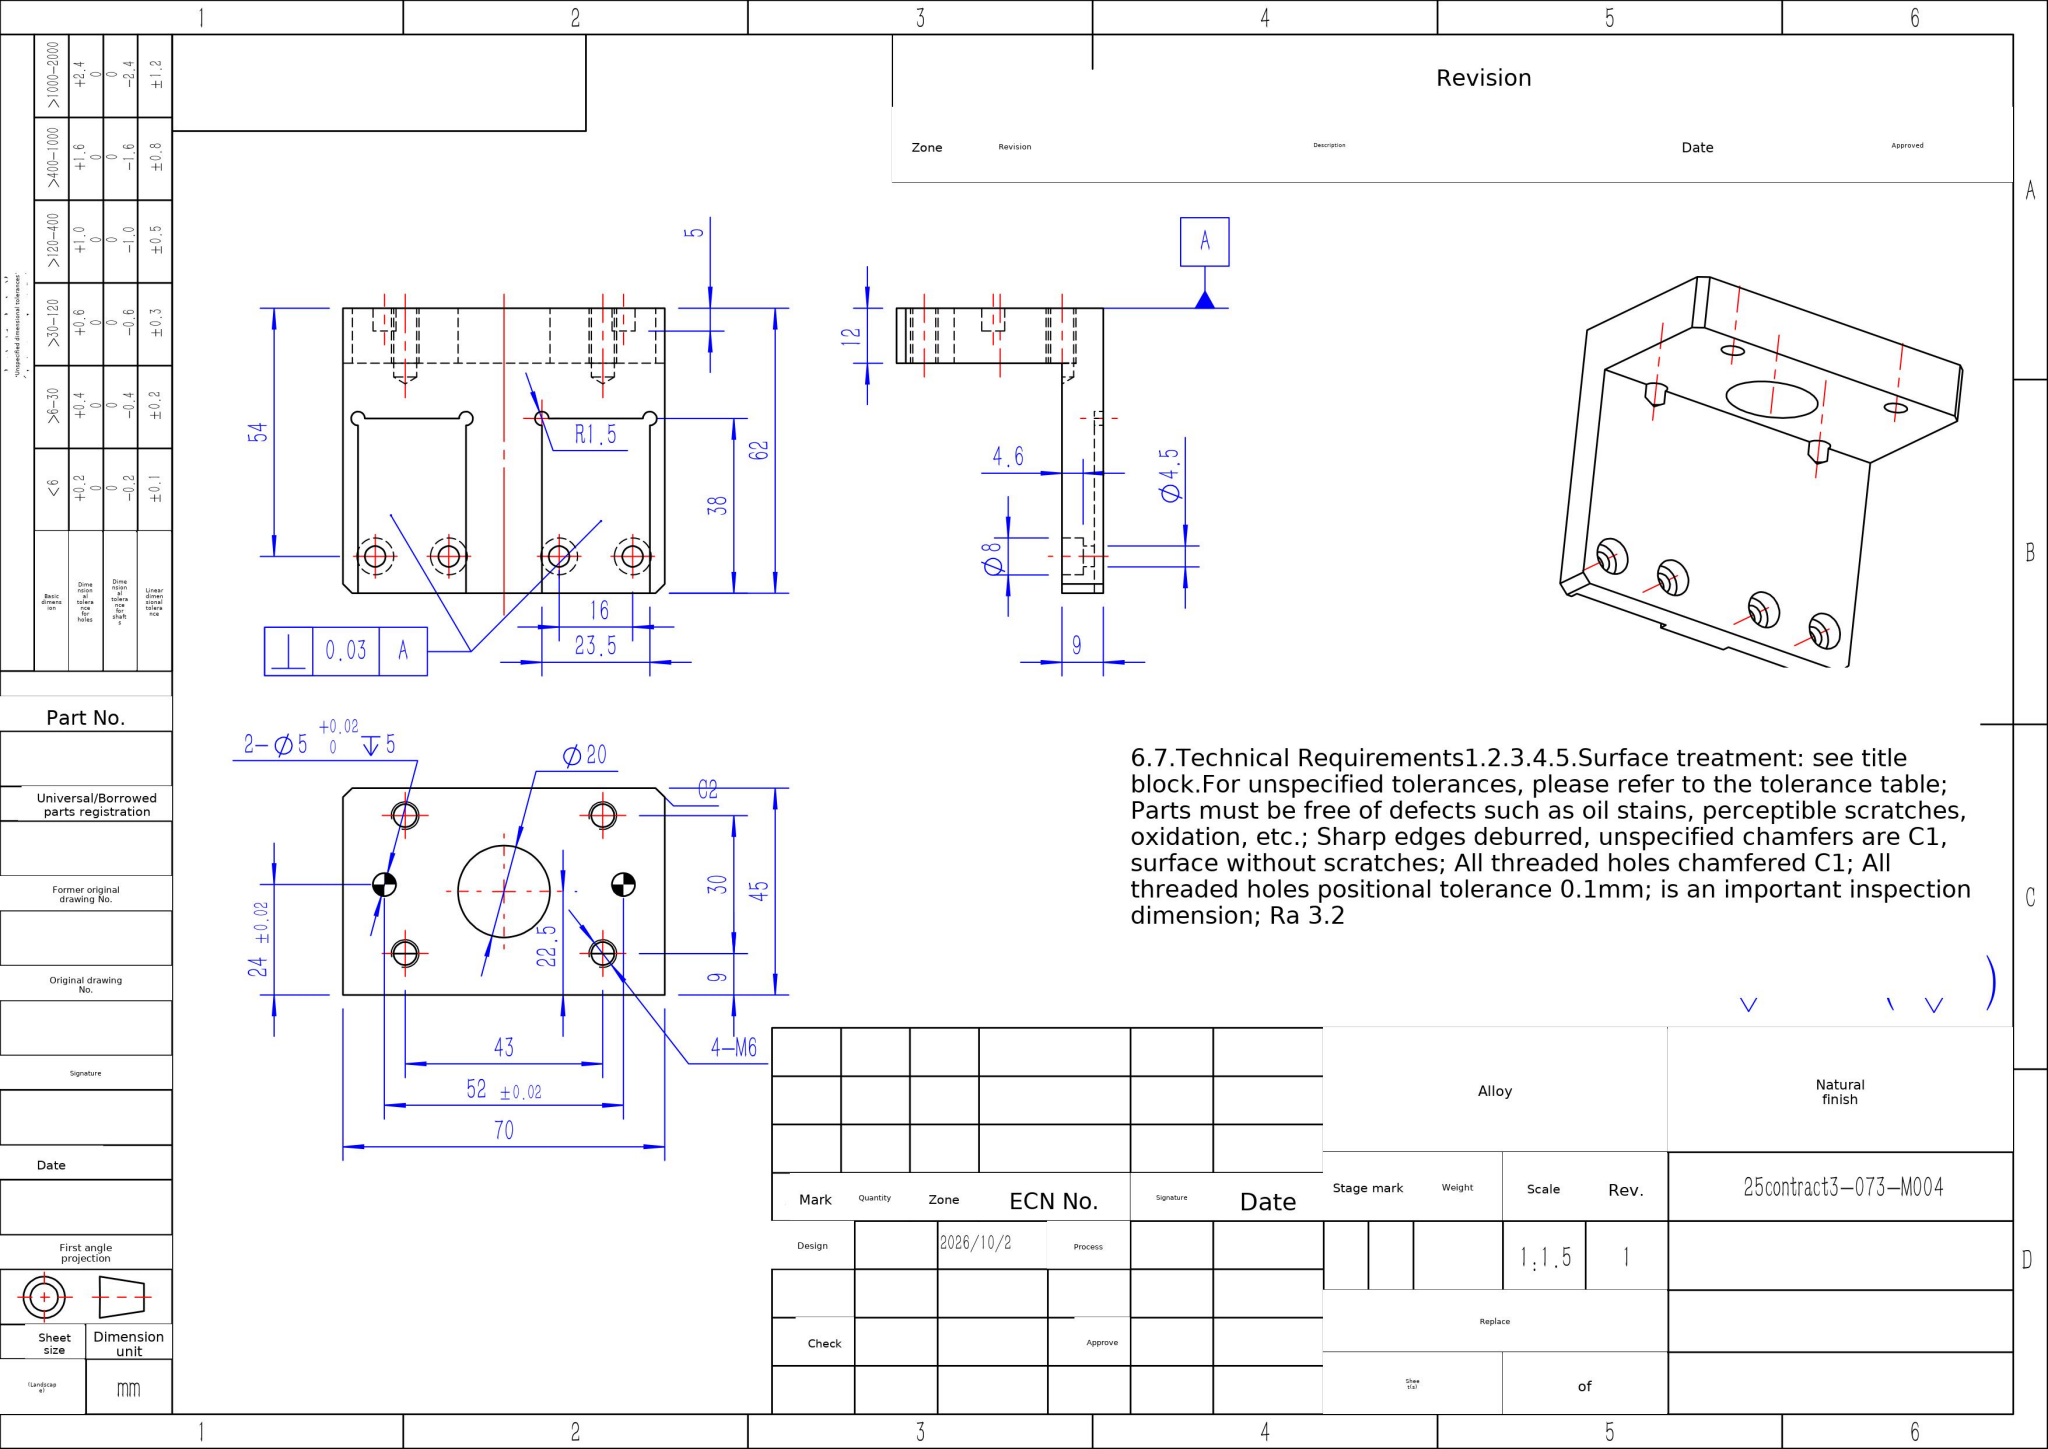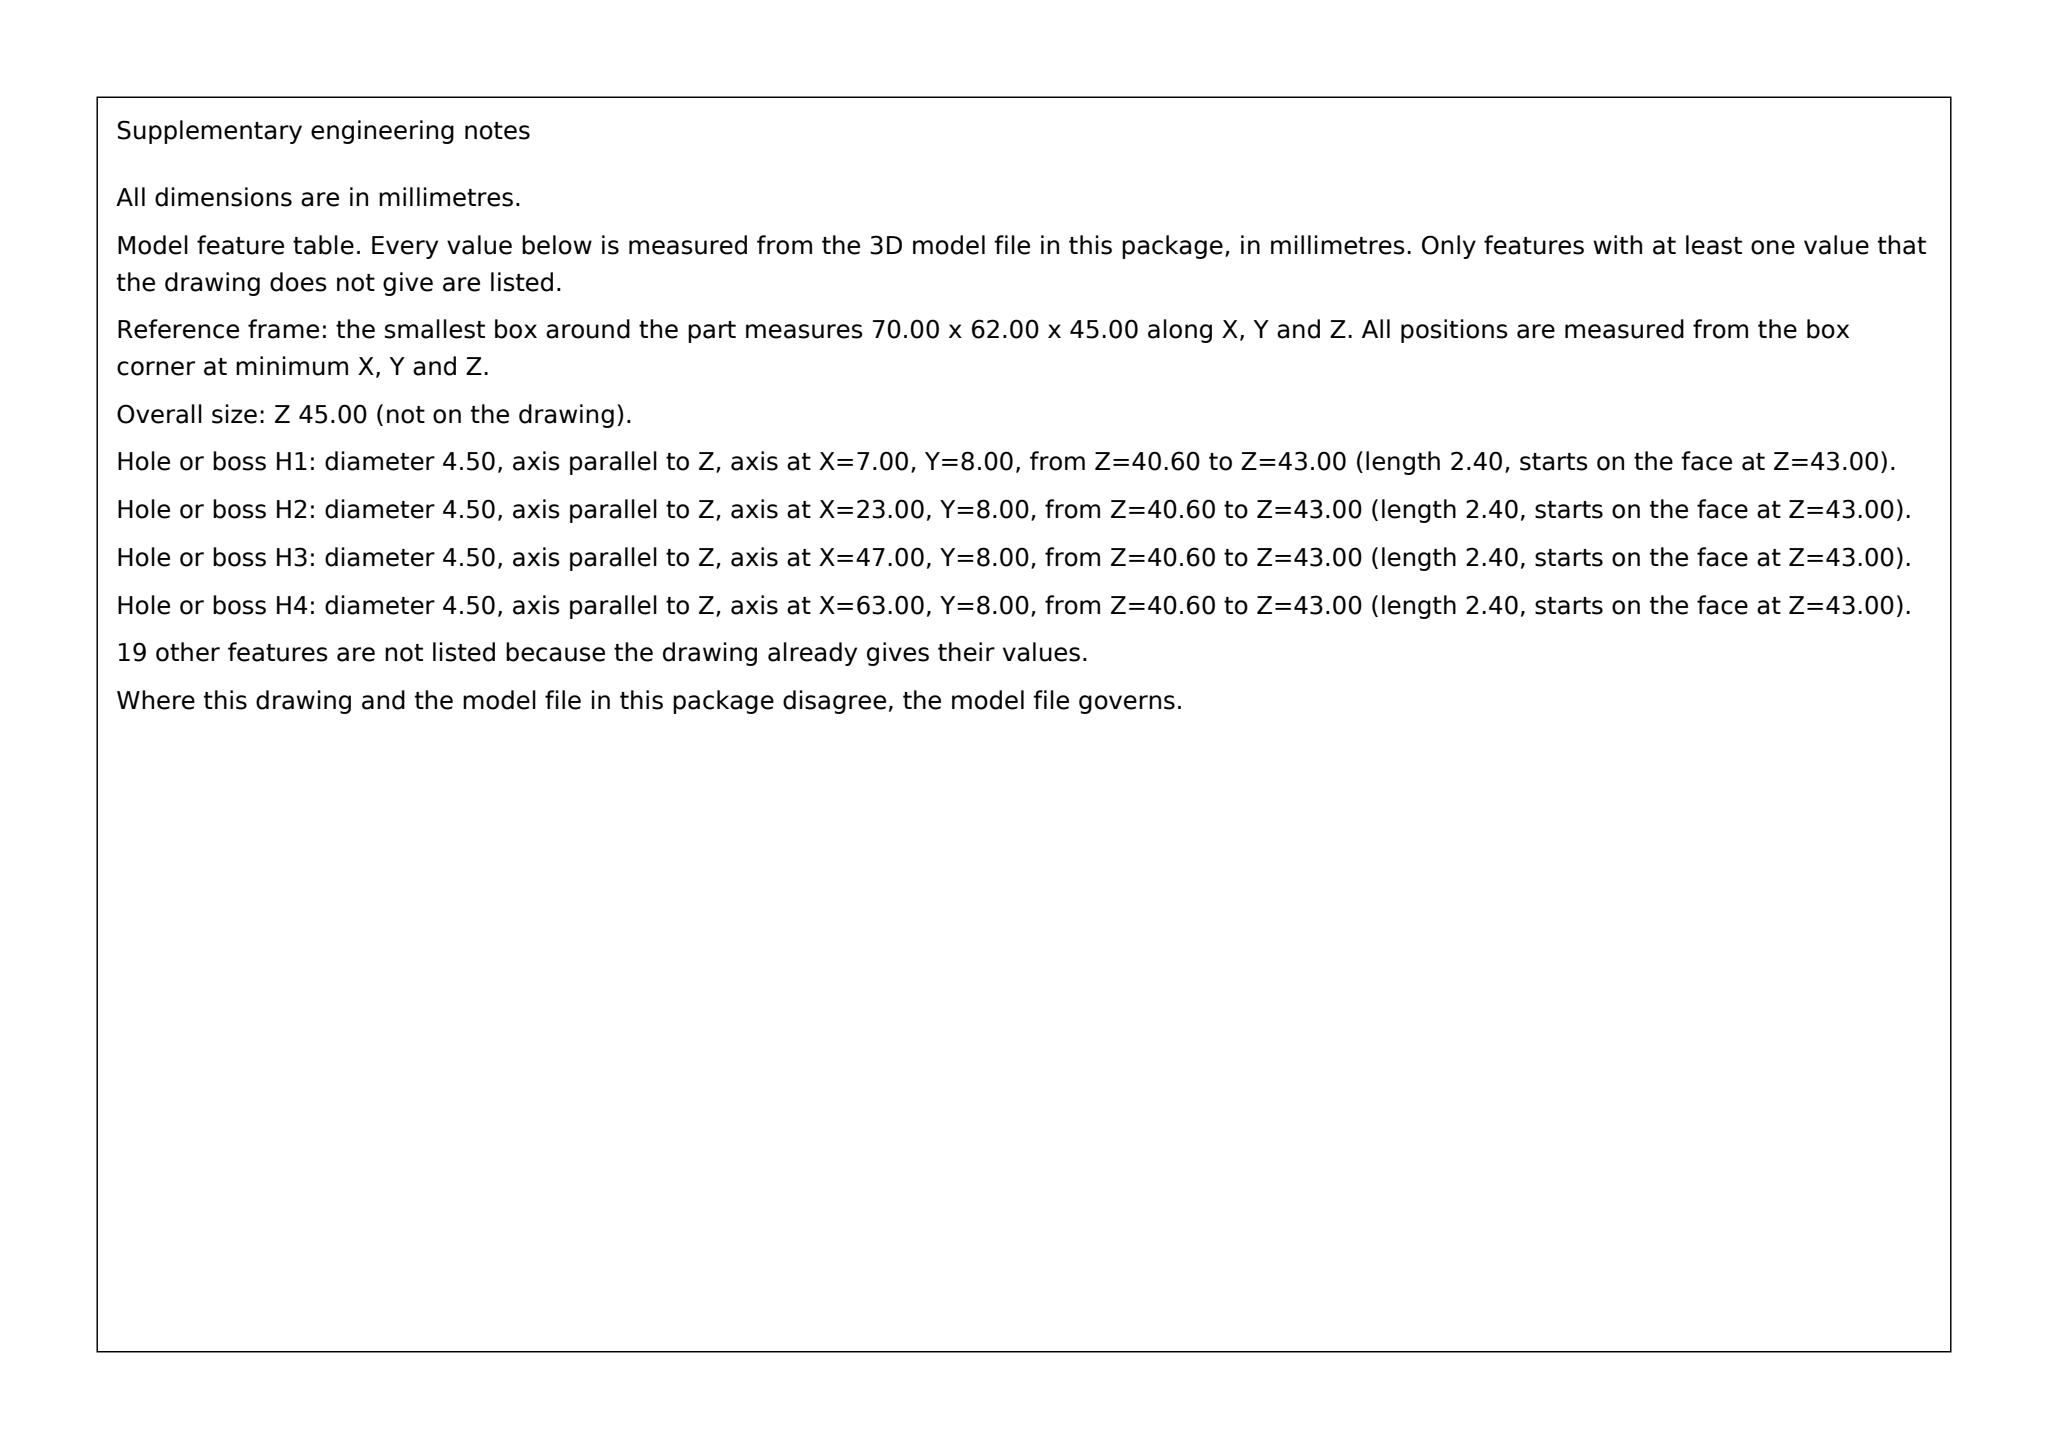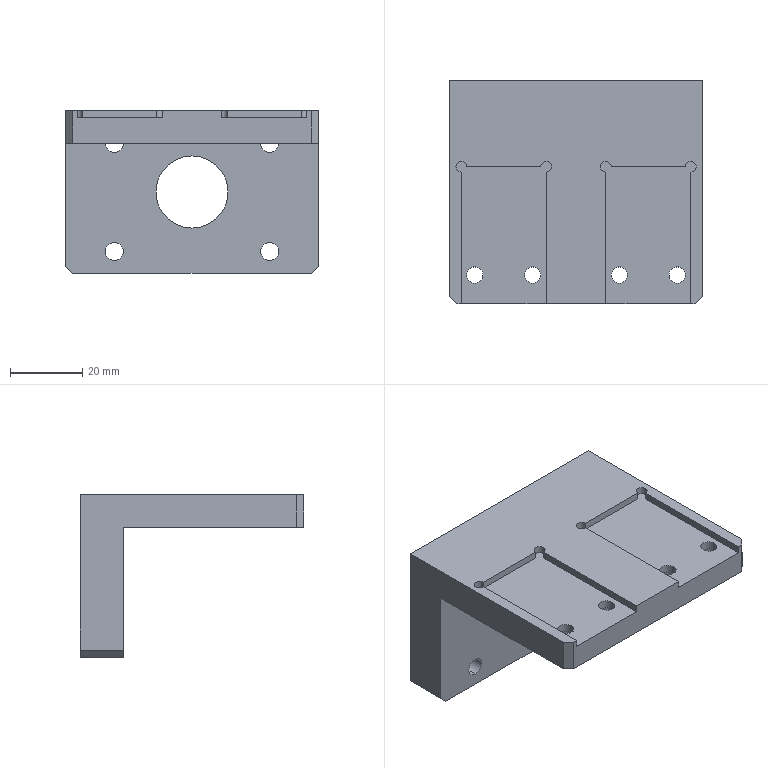Part | SolidWorks | mm | material Alloy | 1 solid | 66 faces | box 70 x 62 x 45 mm | volume 59547 mm3 | cylinder 36 | plane 26 | cone 4 | commonest cylinder face diameters 5 x12 8 x8 4.5 x8 3 x6 20 x2
build123d program:
from build123d import *

# Parameters (mm, degrees)
SKETCH1_W                                         = 110
SKETCH1_H                                         = 45
SKETCH1_R                                         = 10
BOSS_EXTRUDE3_DEPTH                               = 12
SKETCH4_W                                         = 110
SKETCH4_H                                         = 9
BOSS_EXTRUDE4_DEPTH                               = 50
CHAMFER1_SIZE                                     = 5
HOLE_SIZE_ACCORDING_TO_TYPE_1_OF_HEXA_D           = 4.5
HOLE_SIZE_ACCORDING_TO_TYPE_1_OF_HEXA_DEPTH       = 15
HOLE_SIZE_ACCORDING_TO_TYPE_1_OF_HEXA_CBORE_D     = 8
HOLE_SIZE_ACCORDING_TO_TYPE_1_OF_HEXA_CBORE_DEPTH = 4.6
HOLE_SIZE_ACCORDING_TO_TYPE_1_OF_HEXA_TIP         = 1.352
SKETCH10_W                                        = 40.464
SKETCH10_H                                        = 109.227
SKETCH10_W_2                                      = 48.616
SKETCH10_H_2                                      = 131.549
CUT_EXTRUDE1_DEPTH                                = 87.891
CHAMFER2_SIZE                                     = 2
M6_TAPPED_HOLE2_D                                 = 5
M6_TAPPED_HOLE2_DEPTH                             = 15
M6_TAPPED_HOLE2_TIP                               = 1.502
SIZE_MM_DOWEL_PIN_HOLE1_D                         = 5
SIZE_MM_DOWEL_PIN_HOLE1_DEPTH                     = 5
SKETCH19_W                                        = 23.5
SKETCH19_H                                        = 42.5
CUT_EXTRUDE2_DEPTH                                = 2
SKETCH20_R                                        = 1.5
CUT_EXTRUDE3_DEPTH                                = 2


with BuildPart() as part:
    # Sketch1 → Boss-Extrude3 (new body)
    with BuildSketch(Plane(origin=(0, 0, 0), x_dir=(1, 0, 0), z_dir=(0, 1, 0))):
        Rectangle(SKETCH1_W, SKETCH1_H)
        with Locations(Location((0, 0, 0), (0, 0, 270))):
            Circle(SKETCH1_R, mode=Mode.SUBTRACT)
    extrude(amount=BOSS_EXTRUDE3_DEPTH)

    # Sketch4 → Boss-Extrude4 (add)
    with BuildSketch(Plane.XZ):
        with Locations((0, 18)):
            Rectangle(SKETCH4_W, SKETCH4_H)
    extrude(amount=BOSS_EXTRUDE4_DEPTH)

    # Chamfer1
    chamfer1_edges = [part.edges().sort_by_distance(p)[0] for p in [
        (-55, -50, 18),
        (55, -50, 18),
        (-55, 6, -22.5),
        (55, 6, -22.5),
    ]]
    chamfer(chamfer1_edges, length=CHAMFER1_SIZE)

    # Hole Size _ according to_ type 1 of Hexa
    with Locations(Plane(origin=(0, 0, 13.5), x_dir=(-1, 0, 0), z_dir=(0, 0, -1))):
        with Locations((-28, -42), (-12, -42), (12, -42), (28, -42), (-44, -42), (44, -42)):
            CounterBoreHole(HOLE_SIZE_ACCORDING_TO_TYPE_1_OF_HEXA_D / 2, HOLE_SIZE_ACCORDING_TO_TYPE_1_OF_HEXA_CBORE_D / 2, HOLE_SIZE_ACCORDING_TO_TYPE_1_OF_HEXA_CBORE_DEPTH, depth=HOLE_SIZE_ACCORDING_TO_TYPE_1_OF_HEXA_DEPTH)
            with Locations((0, 0, -(HOLE_SIZE_ACCORDING_TO_TYPE_1_OF_HEXA_DEPTH + HOLE_SIZE_ACCORDING_TO_TYPE_1_OF_HEXA_TIP / 2))):  # 118° drill point
                Cone(0, HOLE_SIZE_ACCORDING_TO_TYPE_1_OF_HEXA_D / 2, HOLE_SIZE_ACCORDING_TO_TYPE_1_OF_HEXA_TIP, mode=Mode.SUBTRACT)

    # Sketch10 → Cut-Extrude1 (cut, through all)
    with BuildSketch(Plane.XY.offset(22.5)):
        with Locations((-55.232, -16.021)):
            Rectangle(SKETCH10_W, SKETCH10_H)
        with Locations((59.308, -19.349)):
            Rectangle(SKETCH10_W_2, SKETCH10_H_2)
    extrude(amount=-CUT_EXTRUDE1_DEPTH, mode=Mode.SUBTRACT)

    # Chamfer2
    chamfer2_edges = [part.edges().sort_by_distance(p)[0] for p in [
        (35, -50, 18),
        (-35, -50, 18),
        (-35, 6, -22.5),
        (35, 6, -22.5),
    ]]
    chamfer(chamfer2_edges, length=CHAMFER2_SIZE)

    # M6 Tapped Hole2
    with Locations(Plane(origin=(0, 12, 0), x_dir=(1, 0, 0), z_dir=(0, 1, 0))):
        with Locations((21.5, 16.5), (21.5, -13.5), (-21.5, -13.5), (-21.5, 16.5)):
            Hole(M6_TAPPED_HOLE2_D / 2, depth=M6_TAPPED_HOLE2_DEPTH)
            with Locations((0, 0, -(M6_TAPPED_HOLE2_DEPTH + M6_TAPPED_HOLE2_TIP / 2))):  # 118° drill point
                Cone(0, M6_TAPPED_HOLE2_D / 2, M6_TAPPED_HOLE2_TIP, mode=Mode.SUBTRACT)

    # Size mm Dowel Pin Hole1
    with Locations(Plane(origin=(0, 12, 0), x_dir=(1, 0, 0), z_dir=(0, 1, 0))):
        with Locations((26, 1.5), (-26, 1.5)):
            Hole(SIZE_MM_DOWEL_PIN_HOLE1_D / 2, depth=SIZE_MM_DOWEL_PIN_HOLE1_DEPTH)

    # Sketch19 → Cut-Extrude2 (cut)
    with BuildSketch(Plane.XY.offset(22.5)):
        with Locations((-20, -33.25)):
            Rectangle(SKETCH19_W, SKETCH19_H)
        with Locations((20, -33.25)):
            Rectangle(SKETCH19_W, SKETCH19_H)
    extrude(amount=-CUT_EXTRUDE2_DEPTH, mode=Mode.SUBTRACT)

    # Sketch20 → Cut-Extrude3 (cut)
    with BuildSketch(Plane.XY.offset(20.5)):
        with Locations((-31.75, -12)):
            Circle(SKETCH20_R)
        with Locations((-8.25, -12)):
            Circle(SKETCH20_R)
        with Locations((8.25, -12)):
            Circle(SKETCH20_R)
        with Locations((31.75, -12)):
            Circle(SKETCH20_R)
    extrude(amount=CUT_EXTRUDE3_DEPTH, mode=Mode.SUBTRACT)


solid = part.part